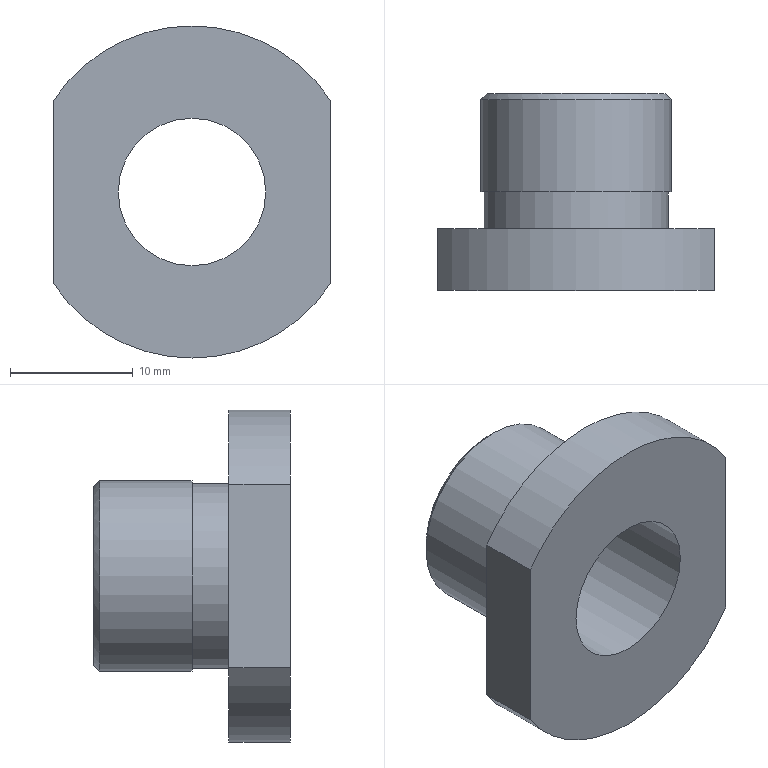Component | NX | CLHKJG_06_THREAD_SEAL_SLEEVE | 1 solid | 13 faces | box 22.5 x 16 x 27 mm | volume 2854 mm3 | plane 6 | cylinder 5 | cone 2 | commonest cylinder face diameters 27 x2 15 x1 15.5 x1 12 x1
STEP:
#1=CARTESIAN_POINT('',(0.,0.,0.));
#2=DIRECTION('',(0.,0.,1.));
#3=DIRECTION('',(1.,0.,0.));
#4=AXIS2_PLACEMENT_3D('',#1,#2,#3);
#5=CARTESIAN_POINT('',(-336.12,36.665,-94.962));
#6=VERTEX_POINT('',#5);
#7=CARTESIAN_POINT('',(-336.12,36.665,-80.038));
#8=VERTEX_POINT('',#7);
#9=CARTESIAN_POINT('',(-336.12,36.665,-94.962));
#10=DIRECTION('',(0.,0.,1.));
#11=VECTOR('',#10,1.);
#12=LINE('',#9,#11);
#13=CARTESIAN_POINT('',(-336.12,31.665,-94.962));
#14=DIRECTION('',(-1.,0.,0.));
#15=DIRECTION('',(0.,0.,1.));
#16=AXIS2_PLACEMENT_3D('',#13,#14,#15);
#17=PLANE('',#16);
#18=CARTESIAN_POINT('',(0.,5.));
#19=DIRECTION('',(1.,0.));
#20=VECTOR('',#19,1.);
#21=LINE('',#18,#20);
#22=(GEOMETRIC_REPRESENTATION_CONTEXT(2)PARAMETRIC_REPRESENTATION_CONTEXT()REPRESENTATION_CONTEXT('',''));
#23=DEFINITIONAL_REPRESENTATION('',(#21),#22);
#24=PCURVE('',#17,#23);
#25=CARTESIAN_POINT('',(-324.87,36.665,-87.5));
#26=DIRECTION('',(0.,1.,0.));
#27=DIRECTION('',(1.,0.,0.));
#28=AXIS2_PLACEMENT_3D('',#25,#26,#27);
#29=PLANE('',#28);
#30=CARTESIAN_POINT('',(-11.25,7.462));
#31=DIRECTION('',(0.,-1.));
#32=VECTOR('',#31,1.);
#33=LINE('',#30,#32);
#34=(GEOMETRIC_REPRESENTATION_CONTEXT(2)PARAMETRIC_REPRESENTATION_CONTEXT()REPRESENTATION_CONTEXT('',''));
#35=DEFINITIONAL_REPRESENTATION('',(#33),#34);
#36=PCURVE('',#29,#35);
#37=SURFACE_CURVE('',#12,(#24,#36),.PCURVE_S1.);
#38=EDGE_CURVE('',#6,#8,#37,.T.);
#39=ORIENTED_EDGE('',*,*,#38,.F.);
#40=CARTESIAN_POINT('',(-336.12,31.665,-94.962));
#41=VERTEX_POINT('',#40);
#42=CARTESIAN_POINT('',(-336.12,31.665,-94.962));
#43=DIRECTION('',(0.,1.,0.));
#44=VECTOR('',#43,1.);
#45=LINE('',#42,#44);
#46=CARTESIAN_POINT('',(0.,0.));
#47=DIRECTION('',(0.,1.));
#48=VECTOR('',#47,1.);
#49=LINE('',#46,#48);
#50=(GEOMETRIC_REPRESENTATION_CONTEXT(2)PARAMETRIC_REPRESENTATION_CONTEXT()REPRESENTATION_CONTEXT('',''));
#51=DEFINITIONAL_REPRESENTATION('',(#49),#50);
#52=PCURVE('',#17,#51);
#53=CARTESIAN_POINT('',(-324.87,31.665,-87.5));
#54=DIRECTION('',(0.,1.,0.));
#55=DIRECTION('',(1.,0.,0.));
#56=AXIS2_PLACEMENT_3D('',#53,#54,#55);
#57=CYLINDRICAL_SURFACE('',#56,13.5);
#58=CARTESIAN_POINT('',(2.556,0.));
#59=DIRECTION('',(0.,1.));
#60=VECTOR('',#59,1.);
#61=LINE('',#58,#60);
#62=(GEOMETRIC_REPRESENTATION_CONTEXT(2)PARAMETRIC_REPRESENTATION_CONTEXT()REPRESENTATION_CONTEXT('',''));
#63=DEFINITIONAL_REPRESENTATION('',(#61),#62);
#64=PCURVE('',#57,#63);
#65=SURFACE_CURVE('',#45,(#52,#64),.PCURVE_S1.);
#66=EDGE_CURVE('',#41,#6,#65,.T.);
#67=ORIENTED_EDGE('',*,*,#66,.F.);
#68=CARTESIAN_POINT('',(-336.12,31.665,-80.038));
#69=VERTEX_POINT('',#68);
#70=CARTESIAN_POINT('',(-336.12,31.665,-94.962));
#71=DIRECTION('',(0.,0.,1.));
#72=VECTOR('',#71,1.);
#73=LINE('',#70,#72);
#74=CARTESIAN_POINT('',(0.,0.));
#75=DIRECTION('',(1.,0.));
#76=VECTOR('',#75,1.);
#77=LINE('',#74,#76);
#78=(GEOMETRIC_REPRESENTATION_CONTEXT(2)PARAMETRIC_REPRESENTATION_CONTEXT()REPRESENTATION_CONTEXT('',''));
#79=DEFINITIONAL_REPRESENTATION('',(#77),#78);
#80=PCURVE('',#17,#79);
#81=CARTESIAN_POINT('',(-324.87,31.665,-87.5));
#82=DIRECTION('',(0.,1.,0.));
#83=DIRECTION('',(1.,0.,0.));
#84=AXIS2_PLACEMENT_3D('',#81,#82,#83);
#85=PLANE('',#84);
#86=CARTESIAN_POINT('',(-11.25,7.462));
#87=DIRECTION('',(0.,-1.));
#88=VECTOR('',#87,1.);
#89=LINE('',#86,#88);
#90=(GEOMETRIC_REPRESENTATION_CONTEXT(2)PARAMETRIC_REPRESENTATION_CONTEXT()REPRESENTATION_CONTEXT('',''));
#91=DEFINITIONAL_REPRESENTATION('',(#89),#90);
#92=PCURVE('',#85,#91);
#93=SURFACE_CURVE('',#73,(#80,#92),.PCURVE_S1.);
#94=EDGE_CURVE('',#41,#69,#93,.T.);
#95=ORIENTED_EDGE('',*,*,#94,.T.);
#96=CARTESIAN_POINT('',(-336.12,31.665,-80.038));
#97=DIRECTION('',(0.,1.,0.));
#98=VECTOR('',#97,1.);
#99=LINE('',#96,#98);
#100=CARTESIAN_POINT('',(14.925,0.));
#101=DIRECTION('',(0.,1.));
#102=VECTOR('',#101,1.);
#103=LINE('',#100,#102);
#104=(GEOMETRIC_REPRESENTATION_CONTEXT(2)PARAMETRIC_REPRESENTATION_CONTEXT()REPRESENTATION_CONTEXT('',''));
#105=DEFINITIONAL_REPRESENTATION('',(#103),#104);
#106=PCURVE('',#17,#105);
#107=CARTESIAN_POINT('',(-324.87,31.665,-87.5));
#108=DIRECTION('',(0.,1.,0.));
#109=DIRECTION('',(1.,0.,0.));
#110=AXIS2_PLACEMENT_3D('',#107,#108,#109);
#111=CYLINDRICAL_SURFACE('',#110,13.5);
#112=CARTESIAN_POINT('',(3.727,0.));
#113=DIRECTION('',(0.,1.));
#114=VECTOR('',#113,1.);
#115=LINE('',#112,#114);
#116=(GEOMETRIC_REPRESENTATION_CONTEXT(2)PARAMETRIC_REPRESENTATION_CONTEXT()REPRESENTATION_CONTEXT('',''));
#117=DEFINITIONAL_REPRESENTATION('',(#115),#116);
#118=PCURVE('',#111,#117);
#119=SURFACE_CURVE('',#99,(#106,#118),.PCURVE_S1.);
#120=EDGE_CURVE('',#69,#8,#119,.T.);
#121=ORIENTED_EDGE('',*,*,#120,.T.);
#122=EDGE_LOOP('',(#39,#67,#95,#121));
#123=FACE_BOUND('',#122,.T.);
#124=ADVANCED_FACE('',(#123),#17,.T.);
#125=CARTESIAN_POINT('',(-313.62,36.665,-80.038));
#126=VERTEX_POINT('',#125);
#127=CARTESIAN_POINT('',(-324.87,36.665,-87.5));
#128=DIRECTION('',(0.,1.,0.));
#129=DIRECTION('',(1.,0.,0.));
#130=AXIS2_PLACEMENT_3D('',#127,#128,#129);
#131=CIRCLE('',#130,13.5);
#132=CARTESIAN_POINT('',(0.,5.));
#133=DIRECTION('',(1.,0.));
#134=VECTOR('',#133,1.);
#135=LINE('',#132,#134);
#136=(GEOMETRIC_REPRESENTATION_CONTEXT(2)PARAMETRIC_REPRESENTATION_CONTEXT()REPRESENTATION_CONTEXT('',''));
#137=DEFINITIONAL_REPRESENTATION('',(#135),#136);
#138=PCURVE('',#111,#137);
#139=CARTESIAN_POINT('',(0.,0.));
#140=DIRECTION('',(1.,0.));
#141=AXIS2_PLACEMENT_2D('',#139,#140);
#142=CIRCLE('',#141,13.5);
#143=(GEOMETRIC_REPRESENTATION_CONTEXT(2)PARAMETRIC_REPRESENTATION_CONTEXT()REPRESENTATION_CONTEXT('',''));
#144=DEFINITIONAL_REPRESENTATION('',(#142),#143);
#145=PCURVE('',#29,#144);
#146=SURFACE_CURVE('',#131,(#138,#145),.PCURVE_S1.);
#147=EDGE_CURVE('',#8,#126,#146,.T.);
#148=ORIENTED_EDGE('',*,*,#147,.F.);
#149=ORIENTED_EDGE('',*,*,#120,.F.);
#150=CARTESIAN_POINT('',(-313.62,31.665,-80.038));
#151=VERTEX_POINT('',#150);
#152=CARTESIAN_POINT('',(-324.87,31.665,-87.5));
#153=DIRECTION('',(0.,1.,0.));
#154=DIRECTION('',(1.,0.,0.));
#155=AXIS2_PLACEMENT_3D('',#152,#153,#154);
#156=CIRCLE('',#155,13.5);
#157=CARTESIAN_POINT('',(0.,0.));
#158=DIRECTION('',(1.,0.));
#159=VECTOR('',#158,1.);
#160=LINE('',#157,#159);
#161=(GEOMETRIC_REPRESENTATION_CONTEXT(2)PARAMETRIC_REPRESENTATION_CONTEXT()REPRESENTATION_CONTEXT('',''));
#162=DEFINITIONAL_REPRESENTATION('',(#160),#161);
#163=PCURVE('',#111,#162);
#164=CARTESIAN_POINT('',(0.,0.));
#165=DIRECTION('',(1.,0.));
#166=AXIS2_PLACEMENT_2D('',#164,#165);
#167=CIRCLE('',#166,13.5);
#168=(GEOMETRIC_REPRESENTATION_CONTEXT(2)PARAMETRIC_REPRESENTATION_CONTEXT()REPRESENTATION_CONTEXT('',''));
#169=DEFINITIONAL_REPRESENTATION('',(#167),#168);
#170=PCURVE('',#85,#169);
#171=SURFACE_CURVE('',#156,(#163,#170),.PCURVE_S1.);
#172=EDGE_CURVE('',#69,#151,#171,.T.);
#173=ORIENTED_EDGE('',*,*,#172,.T.);
#174=CARTESIAN_POINT('',(-313.62,31.665,-80.038));
#175=DIRECTION('',(0.,1.,0.));
#176=VECTOR('',#175,1.);
#177=LINE('',#174,#176);
#178=CARTESIAN_POINT('',(5.697,0.));
#179=DIRECTION('',(0.,1.));
#180=VECTOR('',#179,1.);
#181=LINE('',#178,#180);
#182=(GEOMETRIC_REPRESENTATION_CONTEXT(2)PARAMETRIC_REPRESENTATION_CONTEXT()REPRESENTATION_CONTEXT('',''));
#183=DEFINITIONAL_REPRESENTATION('',(#181),#182);
#184=PCURVE('',#111,#183);
#185=CARTESIAN_POINT('',(-313.62,31.665,-80.038));
#186=DIRECTION('',(1.,0.,0.));
#187=DIRECTION('',(0.,0.,-1.));
#188=AXIS2_PLACEMENT_3D('',#185,#186,#187);
#189=PLANE('',#188);
#190=CARTESIAN_POINT('',(0.,0.));
#191=DIRECTION('',(0.,1.));
#192=VECTOR('',#191,1.);
#193=LINE('',#190,#192);
#194=(GEOMETRIC_REPRESENTATION_CONTEXT(2)PARAMETRIC_REPRESENTATION_CONTEXT()REPRESENTATION_CONTEXT('',''));
#195=DEFINITIONAL_REPRESENTATION('',(#193),#194);
#196=PCURVE('',#189,#195);
#197=SURFACE_CURVE('',#177,(#184,#196),.PCURVE_S1.);
#198=EDGE_CURVE('',#151,#126,#197,.T.);
#199=ORIENTED_EDGE('',*,*,#198,.T.);
#200=EDGE_LOOP('',(#148,#149,#173,#199));
#201=FACE_BOUND('',#200,.T.);
#202=ADVANCED_FACE('',(#201),#111,.T.);
#203=CARTESIAN_POINT('',(-313.62,36.665,-94.962));
#204=VERTEX_POINT('',#203);
#205=CARTESIAN_POINT('',(-313.62,36.665,-80.038));
#206=DIRECTION('',(0.,0.,-1.));
#207=VECTOR('',#206,1.);
#208=LINE('',#205,#207);
#209=CARTESIAN_POINT('',(0.,5.));
#210=DIRECTION('',(1.,0.));
#211=VECTOR('',#210,1.);
#212=LINE('',#209,#211);
#213=(GEOMETRIC_REPRESENTATION_CONTEXT(2)PARAMETRIC_REPRESENTATION_CONTEXT()REPRESENTATION_CONTEXT('',''));
#214=DEFINITIONAL_REPRESENTATION('',(#212),#213);
#215=PCURVE('',#189,#214);
#216=CARTESIAN_POINT('',(11.25,-7.462));
#217=DIRECTION('',(0.,1.));
#218=VECTOR('',#217,1.);
#219=LINE('',#216,#218);
#220=(GEOMETRIC_REPRESENTATION_CONTEXT(2)PARAMETRIC_REPRESENTATION_CONTEXT()REPRESENTATION_CONTEXT('',''));
#221=DEFINITIONAL_REPRESENTATION('',(#219),#220);
#222=PCURVE('',#29,#221);
#223=SURFACE_CURVE('',#208,(#215,#222),.PCURVE_S1.);
#224=EDGE_CURVE('',#126,#204,#223,.T.);
#225=ORIENTED_EDGE('',*,*,#224,.F.);
#226=ORIENTED_EDGE('',*,*,#198,.F.);
#227=CARTESIAN_POINT('',(-313.62,31.665,-94.962));
#228=VERTEX_POINT('',#227);
#229=CARTESIAN_POINT('',(-313.62,31.665,-80.038));
#230=DIRECTION('',(0.,0.,-1.));
#231=VECTOR('',#230,1.);
#232=LINE('',#229,#231);
#233=CARTESIAN_POINT('',(0.,0.));
#234=DIRECTION('',(1.,0.));
#235=VECTOR('',#234,1.);
#236=LINE('',#233,#235);
#237=(GEOMETRIC_REPRESENTATION_CONTEXT(2)PARAMETRIC_REPRESENTATION_CONTEXT()REPRESENTATION_CONTEXT('',''));
#238=DEFINITIONAL_REPRESENTATION('',(#236),#237);
#239=PCURVE('',#189,#238);
#240=CARTESIAN_POINT('',(11.25,-7.462));
#241=DIRECTION('',(0.,1.));
#242=VECTOR('',#241,1.);
#243=LINE('',#240,#242);
#244=(GEOMETRIC_REPRESENTATION_CONTEXT(2)PARAMETRIC_REPRESENTATION_CONTEXT()REPRESENTATION_CONTEXT('',''));
#245=DEFINITIONAL_REPRESENTATION('',(#243),#244);
#246=PCURVE('',#85,#245);
#247=SURFACE_CURVE('',#232,(#239,#246),.PCURVE_S1.);
#248=EDGE_CURVE('',#151,#228,#247,.T.);
#249=ORIENTED_EDGE('',*,*,#248,.T.);
#250=CARTESIAN_POINT('',(-313.62,31.665,-94.962));
#251=DIRECTION('',(0.,1.,0.));
#252=VECTOR('',#251,1.);
#253=LINE('',#250,#252);
#254=CARTESIAN_POINT('',(14.925,0.));
#255=DIRECTION('',(0.,1.));
#256=VECTOR('',#255,1.);
#257=LINE('',#254,#256);
#258=(GEOMETRIC_REPRESENTATION_CONTEXT(2)PARAMETRIC_REPRESENTATION_CONTEXT()REPRESENTATION_CONTEXT('',''));
#259=DEFINITIONAL_REPRESENTATION('',(#257),#258);
#260=PCURVE('',#189,#259);
#261=CARTESIAN_POINT('',(0.5857,0.));
#262=DIRECTION('',(0.,1.));
#263=VECTOR('',#262,1.);
#264=LINE('',#261,#263);
#265=(GEOMETRIC_REPRESENTATION_CONTEXT(2)PARAMETRIC_REPRESENTATION_CONTEXT()REPRESENTATION_CONTEXT('',''));
#266=DEFINITIONAL_REPRESENTATION('',(#264),#265);
#267=PCURVE('',#57,#266);
#268=SURFACE_CURVE('',#253,(#260,#267),.PCURVE_S1.);
#269=EDGE_CURVE('',#228,#204,#268,.T.);
#270=ORIENTED_EDGE('',*,*,#269,.T.);
#271=EDGE_LOOP('',(#225,#226,#249,#270));
#272=FACE_BOUND('',#271,.T.);
#273=ADVANCED_FACE('',(#272),#189,.T.);
#274=CARTESIAN_POINT('',(-324.87,36.665,-87.5));
#275=DIRECTION('',(0.,1.,0.));
#276=DIRECTION('',(1.,0.,0.));
#277=AXIS2_PLACEMENT_3D('',#274,#275,#276);
#278=CIRCLE('',#277,13.5);
#279=CARTESIAN_POINT('',(-0.,5.));
#280=DIRECTION('',(1.,0.));
#281=VECTOR('',#280,1.);
#282=LINE('',#279,#281);
#283=(GEOMETRIC_REPRESENTATION_CONTEXT(2)PARAMETRIC_REPRESENTATION_CONTEXT()REPRESENTATION_CONTEXT('',''));
#284=DEFINITIONAL_REPRESENTATION('',(#282),#283);
#285=PCURVE('',#57,#284);
#286=CARTESIAN_POINT('',(0.,0.));
#287=DIRECTION('',(1.,0.));
#288=AXIS2_PLACEMENT_2D('',#286,#287);
#289=CIRCLE('',#288,13.5);
#290=(GEOMETRIC_REPRESENTATION_CONTEXT(2)PARAMETRIC_REPRESENTATION_CONTEXT()REPRESENTATION_CONTEXT('',''));
#291=DEFINITIONAL_REPRESENTATION('',(#289),#290);
#292=PCURVE('',#29,#291);
#293=SURFACE_CURVE('',#278,(#285,#292),.PCURVE_S1.);
#294=EDGE_CURVE('',#204,#6,#293,.T.);
#295=ORIENTED_EDGE('',*,*,#294,.F.);
#296=ORIENTED_EDGE('',*,*,#269,.F.);
#297=CARTESIAN_POINT('',(-324.87,31.665,-87.5));
#298=DIRECTION('',(0.,1.,0.));
#299=DIRECTION('',(1.,0.,0.));
#300=AXIS2_PLACEMENT_3D('',#297,#298,#299);
#301=CIRCLE('',#300,13.5);
#302=CARTESIAN_POINT('',(-0.,0.));
#303=DIRECTION('',(1.,0.));
#304=VECTOR('',#303,1.);
#305=LINE('',#302,#304);
#306=(GEOMETRIC_REPRESENTATION_CONTEXT(2)PARAMETRIC_REPRESENTATION_CONTEXT()REPRESENTATION_CONTEXT('',''));
#307=DEFINITIONAL_REPRESENTATION('',(#305),#306);
#308=PCURVE('',#57,#307);
#309=CARTESIAN_POINT('',(0.,0.));
#310=DIRECTION('',(1.,0.));
#311=AXIS2_PLACEMENT_2D('',#309,#310);
#312=CIRCLE('',#311,13.5);
#313=(GEOMETRIC_REPRESENTATION_CONTEXT(2)PARAMETRIC_REPRESENTATION_CONTEXT()REPRESENTATION_CONTEXT('',''));
#314=DEFINITIONAL_REPRESENTATION('',(#312),#313);
#315=PCURVE('',#85,#314);
#316=SURFACE_CURVE('',#301,(#308,#315),.PCURVE_S1.);
#317=EDGE_CURVE('',#228,#41,#316,.T.);
#318=ORIENTED_EDGE('',*,*,#317,.T.);
#319=ORIENTED_EDGE('',*,*,#66,.T.);
#320=EDGE_LOOP('',(#295,#296,#318,#319));
#321=FACE_BOUND('',#320,.T.);
#322=ADVANCED_FACE('',(#321),#57,.T.);
#323=CARTESIAN_POINT('',(-318.87,31.665,-87.5));
#324=VERTEX_POINT('',#323);
#325=CARTESIAN_POINT('',(-324.87,31.665,-87.5));
#326=DIRECTION('',(0.,1.,0.));
#327=DIRECTION('',(1.,0.,0.));
#328=AXIS2_PLACEMENT_3D('',#325,#326,#327);
#329=CIRCLE('',#328,6.);
#330=CARTESIAN_POINT('',(0.,0.));
#331=DIRECTION('',(1.,0.));
#332=AXIS2_PLACEMENT_2D('',#330,#331);
#333=CIRCLE('',#332,6.);
#334=(GEOMETRIC_REPRESENTATION_CONTEXT(2)PARAMETRIC_REPRESENTATION_CONTEXT()REPRESENTATION_CONTEXT('',''));
#335=DEFINITIONAL_REPRESENTATION('',(#333),#334);
#336=PCURVE('',#85,#335);
#337=CARTESIAN_POINT('',(-324.87,47.665,-87.5));
#338=DIRECTION('',(0.,-1.,0.));
#339=DIRECTION('',(1.,0.,0.));
#340=AXIS2_PLACEMENT_3D('',#337,#338,#339);
#341=CYLINDRICAL_SURFACE('',#340,6.);
#342=CARTESIAN_POINT('',(6.283,16.));
#343=DIRECTION('',(-1.,0.));
#344=VECTOR('',#343,1.);
#345=LINE('',#342,#344);
#346=(GEOMETRIC_REPRESENTATION_CONTEXT(2)PARAMETRIC_REPRESENTATION_CONTEXT()REPRESENTATION_CONTEXT('',''));
#347=DEFINITIONAL_REPRESENTATION('',(#345),#346);
#348=PCURVE('',#341,#347);
#349=SURFACE_CURVE('',#329,(#336,#348),.PCURVE_S1.);
#350=EDGE_CURVE('',#324,#324,#349,.T.);
#351=ORIENTED_EDGE('',*,*,#350,.T.);
#352=EDGE_LOOP('',(#351));
#353=FACE_BOUND('',#352,.T.);
#354=ORIENTED_EDGE('',*,*,#94,.F.);
#355=ORIENTED_EDGE('',*,*,#317,.F.);
#356=ORIENTED_EDGE('',*,*,#248,.F.);
#357=ORIENTED_EDGE('',*,*,#172,.F.);
#358=EDGE_LOOP('',(#354,#355,#356,#357));
#359=FACE_BOUND('',#358,.T.);
#360=ADVANCED_FACE('',(#353,#359),#85,.F.);
#361=CARTESIAN_POINT('',(-317.37,36.665,-87.5));
#362=VERTEX_POINT('',#361);
#363=CARTESIAN_POINT('',(-324.87,36.665,-87.5));
#364=DIRECTION('',(0.,1.,0.));
#365=DIRECTION('',(1.,0.,0.));
#366=AXIS2_PLACEMENT_3D('',#363,#364,#365);
#367=CIRCLE('',#366,7.5);
#368=CARTESIAN_POINT('',(0.,0.));
#369=DIRECTION('',(1.,0.));
#370=AXIS2_PLACEMENT_2D('',#368,#369);
#371=CIRCLE('',#370,7.5);
#372=(GEOMETRIC_REPRESENTATION_CONTEXT(2)PARAMETRIC_REPRESENTATION_CONTEXT()REPRESENTATION_CONTEXT('',''));
#373=DEFINITIONAL_REPRESENTATION('',(#371),#372);
#374=PCURVE('',#29,#373);
#375=CARTESIAN_POINT('',(-324.87,36.665,-87.5));
#376=DIRECTION('',(0.,1.,0.));
#377=DIRECTION('',(1.,0.,0.));
#378=AXIS2_PLACEMENT_3D('',#375,#376,#377);
#379=CYLINDRICAL_SURFACE('',#378,7.5);
#380=CARTESIAN_POINT('',(0.,0.));
#381=DIRECTION('',(1.,0.));
#382=VECTOR('',#381,1.);
#383=LINE('',#380,#382);
#384=(GEOMETRIC_REPRESENTATION_CONTEXT(2)PARAMETRIC_REPRESENTATION_CONTEXT()REPRESENTATION_CONTEXT('',''));
#385=DEFINITIONAL_REPRESENTATION('',(#383),#384);
#386=PCURVE('',#379,#385);
#387=SURFACE_CURVE('',#367,(#374,#386),.PCURVE_S1.);
#388=EDGE_CURVE('',#362,#362,#387,.T.);
#389=ORIENTED_EDGE('',*,*,#388,.F.);
#390=EDGE_LOOP('',(#389));
#391=FACE_BOUND('',#390,.T.);
#392=ORIENTED_EDGE('',*,*,#38,.T.);
#393=ORIENTED_EDGE('',*,*,#147,.T.);
#394=ORIENTED_EDGE('',*,*,#224,.T.);
#395=ORIENTED_EDGE('',*,*,#294,.T.);
#396=EDGE_LOOP('',(#392,#393,#394,#395));
#397=FACE_BOUND('',#396,.T.);
#398=ADVANCED_FACE('',(#391,#397),#29,.T.);
#399=CARTESIAN_POINT('',(-317.37,39.665,-87.5));
#400=VERTEX_POINT('',#399);
#401=CARTESIAN_POINT('',(-324.87,39.665,-87.5));
#402=DIRECTION('',(0.,-1.,0.));
#403=DIRECTION('',(1.,0.,0.));
#404=AXIS2_PLACEMENT_3D('',#401,#402,#403);
#405=CIRCLE('',#404,7.5);
#406=CARTESIAN_POINT('',(6.283,3.));
#407=DIRECTION('',(-1.,0.));
#408=VECTOR('',#407,1.);
#409=LINE('',#406,#408);
#410=(GEOMETRIC_REPRESENTATION_CONTEXT(2)PARAMETRIC_REPRESENTATION_CONTEXT()REPRESENTATION_CONTEXT('',''));
#411=DEFINITIONAL_REPRESENTATION('',(#409),#410);
#412=PCURVE('',#379,#411);
#413=CARTESIAN_POINT('',(-324.87,39.665,-87.5));
#414=DIRECTION('',(0.,-1.,0.));
#415=DIRECTION('',(-1.,0.,0.));
#416=AXIS2_PLACEMENT_3D('',#413,#414,#415);
#417=PLANE('',#416);
#418=CARTESIAN_POINT('',(0.,0.));
#419=DIRECTION('',(-1.,0.));
#420=AXIS2_PLACEMENT_2D('',#418,#419);
#421=CIRCLE('',#420,7.5);
#422=(GEOMETRIC_REPRESENTATION_CONTEXT(2)PARAMETRIC_REPRESENTATION_CONTEXT()REPRESENTATION_CONTEXT('',''));
#423=DEFINITIONAL_REPRESENTATION('',(#421),#422);
#424=PCURVE('',#417,#423);
#425=SURFACE_CURVE('',#405,(#412,#424),.PCURVE_S1.);
#426=EDGE_CURVE('',#400,#400,#425,.T.);
#427=ORIENTED_EDGE('',*,*,#426,.T.);
#428=CARTESIAN_POINT('',(-317.37,36.665,-87.5));
#429=CARTESIAN_POINT('',(-317.37,39.665,-87.5));
#430=B_SPLINE_CURVE_WITH_KNOTS('',1,(#428,#429),.UNSPECIFIED.,.F.,.F.,(2,2),(0.,3.),.PIECEWISE_BEZIER_KNOTS.);
#431=CARTESIAN_POINT('',(0.,0.));
#432=DIRECTION('',(0.,1.));
#433=VECTOR('',#432,1.);
#434=LINE('',#431,#433);
#435=(GEOMETRIC_REPRESENTATION_CONTEXT(2)PARAMETRIC_REPRESENTATION_CONTEXT()REPRESENTATION_CONTEXT('',''));
#436=DEFINITIONAL_REPRESENTATION('',(#434),#435);
#437=PCURVE('',#379,#436);
#438=CARTESIAN_POINT('',(6.283,0.));
#439=DIRECTION('',(0.,1.));
#440=VECTOR('',#439,1.);
#441=LINE('',#438,#440);
#442=(GEOMETRIC_REPRESENTATION_CONTEXT(2)PARAMETRIC_REPRESENTATION_CONTEXT()REPRESENTATION_CONTEXT('',''));
#443=DEFINITIONAL_REPRESENTATION('',(#441),#442);
#444=PCURVE('',#379,#443);
#445=SEAM_CURVE('',#430,(#437,#444),.PCURVE_S1.);
#446=EDGE_CURVE('',#362,#400,#445,.T.);
#447=ORIENTED_EDGE('',*,*,#446,.F.);
#448=ORIENTED_EDGE('',*,*,#388,.T.);
#449=ORIENTED_EDGE('',*,*,#446,.T.);
#450=EDGE_LOOP('',(#427,#447,#448,#449));
#451=FACE_BOUND('',#450,.T.);
#452=ADVANCED_FACE('',(#451),#379,.T.);
#453=CARTESIAN_POINT('',(-317.62,47.665,-87.5));
#454=VERTEX_POINT('',#453);
#455=CARTESIAN_POINT('',(-324.87,47.665,-87.5));
#456=DIRECTION('',(0.,1.,0.));
#457=DIRECTION('',(1.,0.,0.));
#458=AXIS2_PLACEMENT_3D('',#455,#456,#457);
#459=CIRCLE('',#458,7.25);
#460=CARTESIAN_POINT('',(-324.87,47.665,-87.5));
#461=DIRECTION('',(0.,1.,0.));
#462=DIRECTION('',(1.,0.,0.));
#463=AXIS2_PLACEMENT_3D('',#460,#461,#462);
#464=PLANE('',#463);
#465=CARTESIAN_POINT('',(0.,0.));
#466=DIRECTION('',(1.,0.));
#467=AXIS2_PLACEMENT_2D('',#465,#466);
#468=CIRCLE('',#467,7.25);
#469=(GEOMETRIC_REPRESENTATION_CONTEXT(2)PARAMETRIC_REPRESENTATION_CONTEXT()REPRESENTATION_CONTEXT('',''));
#470=DEFINITIONAL_REPRESENTATION('',(#468),#469);
#471=PCURVE('',#464,#470);
#472=CARTESIAN_POINT('',(-324.87,47.165,-87.5));
#473=DIRECTION('',(0.,-1.,0.));
#474=DIRECTION('',(-1.,0.,0.));
#475=AXIS2_PLACEMENT_3D('',#472,#473,#474);
#476=CONICAL_SURFACE('',#475,7.75,0.7854);
#477=CARTESIAN_POINT('',(9.425,-0.5));
#478=DIRECTION('',(-1.,0.));
#479=VECTOR('',#478,1.);
#480=LINE('',#477,#479);
#481=(GEOMETRIC_REPRESENTATION_CONTEXT(2)PARAMETRIC_REPRESENTATION_CONTEXT()REPRESENTATION_CONTEXT('',''));
#482=DEFINITIONAL_REPRESENTATION('',(#480),#481);
#483=PCURVE('',#476,#482);
#484=SURFACE_CURVE('',#459,(#471,#483),.PCURVE_S1.);
#485=EDGE_CURVE('',#454,#454,#484,.T.);
#486=ORIENTED_EDGE('',*,*,#485,.T.);
#487=EDGE_LOOP('',(#486));
#488=FACE_BOUND('',#487,.T.);
#489=CARTESIAN_POINT('',(-318.37,47.665,-87.5));
#490=VERTEX_POINT('',#489);
#491=CARTESIAN_POINT('',(-324.87,47.665,-87.5));
#492=DIRECTION('',(0.,-1.,0.));
#493=DIRECTION('',(1.,0.,0.));
#494=AXIS2_PLACEMENT_3D('',#491,#492,#493);
#495=CIRCLE('',#494,6.5);
#496=CARTESIAN_POINT('',(6.5,0.));
#497=CARTESIAN_POINT('',(6.5,-11.258));
#498=CARTESIAN_POINT('',(-3.25,-5.629));
#499=CARTESIAN_POINT('',(-13.,-0.));
#500=CARTESIAN_POINT('',(-3.25,5.629));
#501=CARTESIAN_POINT('',(6.5,11.258));
#502=CARTESIAN_POINT('',(6.5,0.));
#503=(BOUNDED_CURVE()B_SPLINE_CURVE(2,(#496,#497,#498,#499,#500,#501,#502),.UNSPECIFIED.,.T.,.F.)B_SPLINE_CURVE_WITH_KNOTS((1,2,2,2,2,1),(-2.094,0.,2.094,4.189,6.283,8.378),.UNSPECIFIED.)CURVE()GEOMETRIC_REPRESENTATION_ITEM()RATIONAL_B_SPLINE_CURVE((1.,0.5,1.,0.5,1.,0.5,1.))REPRESENTATION_ITEM(''));
#504=(GEOMETRIC_REPRESENTATION_CONTEXT(2)PARAMETRIC_REPRESENTATION_CONTEXT()REPRESENTATION_CONTEXT('',''));
#505=DEFINITIONAL_REPRESENTATION('',(#503),#504);
#506=PCURVE('',#464,#505);
#507=CARTESIAN_POINT('',(-324.87,47.665,-87.5));
#508=DIRECTION('',(0.,1.,0.));
#509=DIRECTION('',(1.,0.,0.));
#510=AXIS2_PLACEMENT_3D('',#507,#508,#509);
#511=CONICAL_SURFACE('',#510,6.5,0.7854);
#512=CARTESIAN_POINT('',(6.283,0.));
#513=DIRECTION('',(-1.,0.));
#514=VECTOR('',#513,1.);
#515=LINE('',#512,#514);
#516=(GEOMETRIC_REPRESENTATION_CONTEXT(2)PARAMETRIC_REPRESENTATION_CONTEXT()REPRESENTATION_CONTEXT('',''));
#517=DEFINITIONAL_REPRESENTATION('',(#515),#516);
#518=PCURVE('',#511,#517);
#519=SURFACE_CURVE('',#495,(#506,#518),.PCURVE_S1.);
#520=EDGE_CURVE('',#490,#490,#519,.T.);
#521=ORIENTED_EDGE('',*,*,#520,.T.);
#522=EDGE_LOOP('',(#521));
#523=FACE_BOUND('',#522,.T.);
#524=ADVANCED_FACE('',(#488,#523),#464,.T.);
#525=ORIENTED_EDGE('',*,*,#426,.F.);
#526=EDGE_LOOP('',(#525));
#527=FACE_BOUND('',#526,.T.);
#528=CARTESIAN_POINT('',(-317.12,39.665,-87.5));
#529=VERTEX_POINT('',#528);
#530=CARTESIAN_POINT('',(-324.87,39.665,-87.5));
#531=DIRECTION('',(0.,1.,0.));
#532=DIRECTION('',(1.,0.,0.));
#533=AXIS2_PLACEMENT_3D('',#530,#531,#532);
#534=CIRCLE('',#533,7.75);
#535=CARTESIAN_POINT('',(-7.75,0.));
#536=CARTESIAN_POINT('',(-7.75,13.423));
#537=CARTESIAN_POINT('',(3.875,6.712));
#538=CARTESIAN_POINT('',(15.5,0.));
#539=CARTESIAN_POINT('',(3.875,-6.712));
#540=CARTESIAN_POINT('',(-7.75,-13.423));
#541=CARTESIAN_POINT('',(-7.75,0.));
#542=(BOUNDED_CURVE()B_SPLINE_CURVE(2,(#535,#536,#537,#538,#539,#540,#541),.UNSPECIFIED.,.T.,.F.)B_SPLINE_CURVE_WITH_KNOTS((1,2,2,2,2,1),(-2.094,0.,2.094,4.189,6.283,8.378),.UNSPECIFIED.)CURVE()GEOMETRIC_REPRESENTATION_ITEM()RATIONAL_B_SPLINE_CURVE((1.,0.5,1.,0.5,1.,0.5,1.))REPRESENTATION_ITEM(''));
#543=(GEOMETRIC_REPRESENTATION_CONTEXT(2)PARAMETRIC_REPRESENTATION_CONTEXT()REPRESENTATION_CONTEXT('',''));
#544=DEFINITIONAL_REPRESENTATION('',(#542),#543);
#545=PCURVE('',#417,#544);
#546=CARTESIAN_POINT('',(-324.87,39.665,-87.5));
#547=DIRECTION('',(0.,1.,0.));
#548=DIRECTION('',(1.,0.,0.));
#549=AXIS2_PLACEMENT_3D('',#546,#547,#548);
#550=CYLINDRICAL_SURFACE('',#549,7.75);
#551=CARTESIAN_POINT('',(0.,0.));
#552=DIRECTION('',(1.,0.));
#553=VECTOR('',#552,1.);
#554=LINE('',#551,#553);
#555=(GEOMETRIC_REPRESENTATION_CONTEXT(2)PARAMETRIC_REPRESENTATION_CONTEXT()REPRESENTATION_CONTEXT('',''));
#556=DEFINITIONAL_REPRESENTATION('',(#554),#555);
#557=PCURVE('',#550,#556);
#558=SURFACE_CURVE('',#534,(#545,#557),.PCURVE_S1.);
#559=EDGE_CURVE('',#529,#529,#558,.T.);
#560=ORIENTED_EDGE('',*,*,#559,.F.);
#561=EDGE_LOOP('',(#560));
#562=FACE_BOUND('',#561,.T.);
#563=ADVANCED_FACE('',(#527,#562),#417,.T.);
#564=CARTESIAN_POINT('',(-317.12,47.165,-87.5));
#565=VERTEX_POINT('',#564);
#566=CARTESIAN_POINT('',(-324.87,47.165,-87.5));
#567=DIRECTION('',(0.,-1.,0.));
#568=DIRECTION('',(1.,0.,0.));
#569=AXIS2_PLACEMENT_3D('',#566,#567,#568);
#570=CIRCLE('',#569,7.75);
#571=CARTESIAN_POINT('',(6.283,7.5));
#572=DIRECTION('',(-1.,0.));
#573=VECTOR('',#572,1.);
#574=LINE('',#571,#573);
#575=(GEOMETRIC_REPRESENTATION_CONTEXT(2)PARAMETRIC_REPRESENTATION_CONTEXT()REPRESENTATION_CONTEXT('',''));
#576=DEFINITIONAL_REPRESENTATION('',(#574),#575);
#577=PCURVE('',#550,#576);
#578=CARTESIAN_POINT('',(3.142,0.));
#579=DIRECTION('',(1.,0.));
#580=VECTOR('',#579,1.);
#581=LINE('',#578,#580);
#582=(GEOMETRIC_REPRESENTATION_CONTEXT(2)PARAMETRIC_REPRESENTATION_CONTEXT()REPRESENTATION_CONTEXT('',''));
#583=DEFINITIONAL_REPRESENTATION('',(#581),#582);
#584=PCURVE('',#476,#583);
#585=SURFACE_CURVE('',#570,(#577,#584),.PCURVE_S1.);
#586=EDGE_CURVE('',#565,#565,#585,.T.);
#587=ORIENTED_EDGE('',*,*,#586,.T.);
#588=CARTESIAN_POINT('',(-317.12,39.665,-87.5));
#589=CARTESIAN_POINT('',(-317.12,47.165,-87.5));
#590=B_SPLINE_CURVE_WITH_KNOTS('',1,(#588,#589),.UNSPECIFIED.,.F.,.F.,(2,2),(0.,7.5),.PIECEWISE_BEZIER_KNOTS.);
#591=CARTESIAN_POINT('',(0.,0.));
#592=DIRECTION('',(0.,1.));
#593=VECTOR('',#592,1.);
#594=LINE('',#591,#593);
#595=(GEOMETRIC_REPRESENTATION_CONTEXT(2)PARAMETRIC_REPRESENTATION_CONTEXT()REPRESENTATION_CONTEXT('',''));
#596=DEFINITIONAL_REPRESENTATION('',(#594),#595);
#597=PCURVE('',#550,#596);
#598=CARTESIAN_POINT('',(6.283,0.));
#599=DIRECTION('',(0.,1.));
#600=VECTOR('',#599,1.);
#601=LINE('',#598,#600);
#602=(GEOMETRIC_REPRESENTATION_CONTEXT(2)PARAMETRIC_REPRESENTATION_CONTEXT()REPRESENTATION_CONTEXT('',''));
#603=DEFINITIONAL_REPRESENTATION('',(#601),#602);
#604=PCURVE('',#550,#603);
#605=SEAM_CURVE('',#590,(#597,#604),.PCURVE_S1.);
#606=EDGE_CURVE('',#529,#565,#605,.T.);
#607=ORIENTED_EDGE('',*,*,#606,.F.);
#608=ORIENTED_EDGE('',*,*,#559,.T.);
#609=ORIENTED_EDGE('',*,*,#606,.T.);
#610=EDGE_LOOP('',(#587,#607,#608,#609));
#611=FACE_BOUND('',#610,.T.);
#612=ADVANCED_FACE('',(#611),#550,.T.);
#613=CARTESIAN_POINT('',(-318.87,47.165,-87.5));
#614=VERTEX_POINT('',#613);
#615=CARTESIAN_POINT('',(-324.87,47.165,-87.5));
#616=DIRECTION('',(0.,1.,0.));
#617=DIRECTION('',(1.,0.,0.));
#618=AXIS2_PLACEMENT_3D('',#615,#616,#617);
#619=CIRCLE('',#618,6.);
#620=CARTESIAN_POINT('',(6.283,0.5));
#621=DIRECTION('',(-1.,0.));
#622=VECTOR('',#621,1.);
#623=LINE('',#620,#622);
#624=(GEOMETRIC_REPRESENTATION_CONTEXT(2)PARAMETRIC_REPRESENTATION_CONTEXT()REPRESENTATION_CONTEXT('',''));
#625=DEFINITIONAL_REPRESENTATION('',(#623),#624);
#626=PCURVE('',#341,#625);
#627=CARTESIAN_POINT('',(0.,-0.5));
#628=DIRECTION('',(1.,0.));
#629=VECTOR('',#628,1.);
#630=LINE('',#627,#629);
#631=(GEOMETRIC_REPRESENTATION_CONTEXT(2)PARAMETRIC_REPRESENTATION_CONTEXT()REPRESENTATION_CONTEXT('',''));
#632=DEFINITIONAL_REPRESENTATION('',(#630),#631);
#633=PCURVE('',#511,#632);
#634=SURFACE_CURVE('',#619,(#626,#633),.PCURVE_S1.);
#635=EDGE_CURVE('',#614,#614,#634,.T.);
#636=ORIENTED_EDGE('',*,*,#635,.F.);
#637=CARTESIAN_POINT('',(-318.87,47.165,-87.5));
#638=CARTESIAN_POINT('',(-318.87,31.665,-87.5));
#639=B_SPLINE_CURVE_WITH_KNOTS('',1,(#637,#638),.UNSPECIFIED.,.F.,.F.,(2,2),(0.5,16.),.PIECEWISE_BEZIER_KNOTS.);
#640=CARTESIAN_POINT('',(6.283,0.));
#641=DIRECTION('',(0.,1.));
#642=VECTOR('',#641,1.);
#643=LINE('',#640,#642);
#644=(GEOMETRIC_REPRESENTATION_CONTEXT(2)PARAMETRIC_REPRESENTATION_CONTEXT()REPRESENTATION_CONTEXT('',''));
#645=DEFINITIONAL_REPRESENTATION('',(#643),#644);
#646=PCURVE('',#341,#645);
#647=CARTESIAN_POINT('',(0.,0.));
#648=DIRECTION('',(0.,1.));
#649=VECTOR('',#648,1.);
#650=LINE('',#647,#649);
#651=(GEOMETRIC_REPRESENTATION_CONTEXT(2)PARAMETRIC_REPRESENTATION_CONTEXT()REPRESENTATION_CONTEXT('',''));
#652=DEFINITIONAL_REPRESENTATION('',(#650),#651);
#653=PCURVE('',#341,#652);
#654=SEAM_CURVE('',#639,(#646,#653),.PCURVE_S1.);
#655=EDGE_CURVE('',#614,#324,#654,.T.);
#656=ORIENTED_EDGE('',*,*,#655,.T.);
#657=ORIENTED_EDGE('',*,*,#350,.T.);
#658=ORIENTED_EDGE('',*,*,#655,.F.);
#659=EDGE_LOOP('',(#636,#656,#657,#658));
#660=FACE_BOUND('',#659,.F.);
#661=ADVANCED_FACE('',(#660),#341,.F.);
#662=ORIENTED_EDGE('',*,*,#485,.F.);
#663=CARTESIAN_POINT('',(-317.62,47.665,-87.5));
#664=CARTESIAN_POINT('',(-317.12,47.165,-87.5));
#665=B_SPLINE_CURVE_WITH_KNOTS('',1,(#663,#664),.UNSPECIFIED.,.F.,.F.,(2,2),(-0.7071,0.),.PIECEWISE_BEZIER_KNOTS.);
#666=CARTESIAN_POINT('',(9.425,0.));
#667=DIRECTION('',(0.,1.));
#668=VECTOR('',#667,1.);
#669=LINE('',#666,#668);
#670=(GEOMETRIC_REPRESENTATION_CONTEXT(2)PARAMETRIC_REPRESENTATION_CONTEXT()REPRESENTATION_CONTEXT('',''));
#671=DEFINITIONAL_REPRESENTATION('',(#669),#670);
#672=PCURVE('',#476,#671);
#673=CARTESIAN_POINT('',(3.142,0.));
#674=DIRECTION('',(0.,1.));
#675=VECTOR('',#674,1.);
#676=LINE('',#673,#675);
#677=(GEOMETRIC_REPRESENTATION_CONTEXT(2)PARAMETRIC_REPRESENTATION_CONTEXT()REPRESENTATION_CONTEXT('',''));
#678=DEFINITIONAL_REPRESENTATION('',(#676),#677);
#679=PCURVE('',#476,#678);
#680=SEAM_CURVE('',#665,(#672,#679),.PCURVE_S1.);
#681=EDGE_CURVE('',#454,#565,#680,.T.);
#682=ORIENTED_EDGE('',*,*,#681,.T.);
#683=ORIENTED_EDGE('',*,*,#586,.F.);
#684=ORIENTED_EDGE('',*,*,#681,.F.);
#685=EDGE_LOOP('',(#662,#682,#683,#684));
#686=FACE_BOUND('',#685,.T.);
#687=ADVANCED_FACE('',(#686),#476,.T.);
#688=ORIENTED_EDGE('',*,*,#635,.T.);
#689=CARTESIAN_POINT('',(-318.87,47.165,-87.5));
#690=CARTESIAN_POINT('',(-318.37,47.665,-87.5));
#691=B_SPLINE_CURVE_WITH_KNOTS('',1,(#689,#690),.UNSPECIFIED.,.F.,.F.,(2,2),(-0.7071,0.),.PIECEWISE_BEZIER_KNOTS.);
#692=CARTESIAN_POINT('',(6.283,0.));
#693=DIRECTION('',(0.,1.));
#694=VECTOR('',#693,1.);
#695=LINE('',#692,#694);
#696=(GEOMETRIC_REPRESENTATION_CONTEXT(2)PARAMETRIC_REPRESENTATION_CONTEXT()REPRESENTATION_CONTEXT('',''));
#697=DEFINITIONAL_REPRESENTATION('',(#695),#696);
#698=PCURVE('',#511,#697);
#699=CARTESIAN_POINT('',(0.,0.));
#700=DIRECTION('',(0.,1.));
#701=VECTOR('',#700,1.);
#702=LINE('',#699,#701);
#703=(GEOMETRIC_REPRESENTATION_CONTEXT(2)PARAMETRIC_REPRESENTATION_CONTEXT()REPRESENTATION_CONTEXT('',''));
#704=DEFINITIONAL_REPRESENTATION('',(#702),#703);
#705=PCURVE('',#511,#704);
#706=SEAM_CURVE('',#691,(#698,#705),.PCURVE_S1.);
#707=EDGE_CURVE('',#614,#490,#706,.T.);
#708=ORIENTED_EDGE('',*,*,#707,.T.);
#709=ORIENTED_EDGE('',*,*,#520,.T.);
#710=ORIENTED_EDGE('',*,*,#707,.F.);
#711=EDGE_LOOP('',(#688,#708,#709,#710));
#712=FACE_BOUND('',#711,.F.);
#713=ADVANCED_FACE('',(#712),#511,.F.);
#714=CLOSED_SHELL('',(#124,#202,#273,#322,#360,#398,#452,#524,#563,#612,#661,#687,#713));
#715=MANIFOLD_SOLID_BREP('',#714);
#716=(LENGTH_UNIT()NAMED_UNIT(*)SI_UNIT(.MILLI.,.METRE.));
#717=UNCERTAINTY_MEASURE_WITH_UNIT(LENGTH_MEASURE(0.000005),#716,'','');
#718=(NAMED_UNIT(*)PLANE_ANGLE_UNIT()SI_UNIT($,.RADIAN.));
#719=(NAMED_UNIT(*)SI_UNIT($,.STERADIAN.)SOLID_ANGLE_UNIT());
#720=(GEOMETRIC_REPRESENTATION_CONTEXT(3)GLOBAL_UNCERTAINTY_ASSIGNED_CONTEXT((#717))GLOBAL_UNIT_ASSIGNED_CONTEXT((#716,#718,#719))REPRESENTATION_CONTEXT('',''));
#721=ADVANCED_BREP_SHAPE_REPRESENTATION('',(#4,#715),#720);